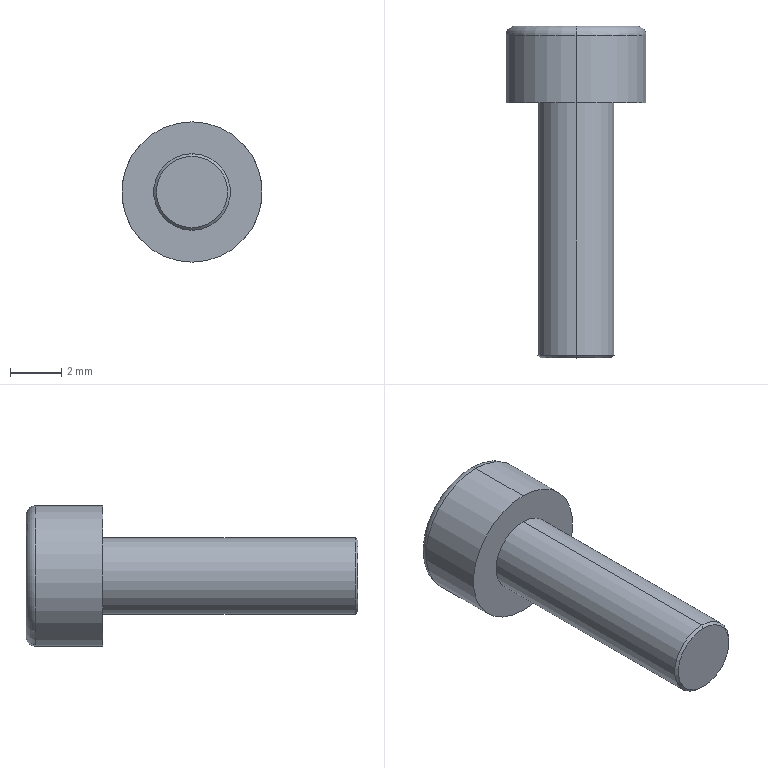Component | SolidWorks | hexagon socket head cap screws gb-1 | 1 solid | 25 faces | box 5.5 x 13 x 5.5 mm | volume 133 mm3 | plane 15 | cone 4 | cylinder 4 | torus 2 | commonest cylinder face diameters 3 x2 5.5 x2
STEP:
#1=CARTESIAN_POINT('',(-3.507,21.249,24.369));
#2=VERTEX_POINT('',#1);
#3=CARTESIAN_POINT('',(-3.507,21.249,24.479));
#4=VERTEX_POINT('',#3);
#5=CARTESIAN_POINT('',(-3.507,21.249,24.424));
#6=DIRECTION('',(0.,-1.,-0.));
#7=DIRECTION('',(0.,0.,-1.));
#8=AXIS2_PLACEMENT_3D('',#5,#6,#7);
#9=CIRCLE('',#8,0.05512);
#10=EDGE_CURVE('',#2,#4,#9,.T.);
#11=ORIENTED_EDGE('',*,*,#10,.F.);
#12=CARTESIAN_POINT('',(-3.507,21.253,24.365));
#13=VERTEX_POINT('',#12);
#14=CARTESIAN_POINT('',(-3.507,21.249,24.369));
#15=DIRECTION('',(-0.,0.7071,-0.7071));
#16=VECTOR('',#15,39.37);
#17=LINE('',#14,#16);
#18=EDGE_CURVE('',#2,#13,#17,.T.);
#19=ORIENTED_EDGE('',*,*,#18,.T.);
#20=CARTESIAN_POINT('',(-3.507,21.253,24.483));
#21=VERTEX_POINT('',#20);
#22=CARTESIAN_POINT('',(-3.507,21.253,24.424));
#23=DIRECTION('',(-0.,1.,0.));
#24=DIRECTION('',(0.,0.,-1.));
#25=AXIS2_PLACEMENT_3D('',#22,#23,#24);
#26=CIRCLE('',#25,0.05906);
#27=EDGE_CURVE('',#21,#13,#26,.T.);
#28=ORIENTED_EDGE('',*,*,#27,.F.);
#29=CARTESIAN_POINT('',(-3.507,21.249,24.479));
#30=DIRECTION('',(0.,0.7071,0.7071));
#31=VECTOR('',#30,39.37);
#32=LINE('',#29,#31);
#33=EDGE_CURVE('',#4,#21,#32,.T.);
#34=ORIENTED_EDGE('',*,*,#33,.F.);
#35=EDGE_LOOP('',(#11,#19,#28,#34));
#36=FACE_OUTER_BOUND('',#35,.T.);
#37=CARTESIAN_POINT('',(-3.507,21.249,24.424));
#38=DIRECTION('',(-0.,1.,0.));
#39=DIRECTION('',(0.,0.,1.));
#40=AXIS2_PLACEMENT_3D('',#37,#38,#39);
#41=CONICAL_SURFACE('',#40,0.05512,0.7854);
#42=ADVANCED_FACE('',(#36),#41,.T.);
#43=CARTESIAN_POINT('',(-3.507,21.761,24.517));
#44=VERTEX_POINT('',#43);
#45=CARTESIAN_POINT('',(-3.507,21.761,24.33));
#46=VERTEX_POINT('',#45);
#47=CARTESIAN_POINT('',(-3.507,21.761,24.424));
#48=DIRECTION('',(-0.,1.,0.));
#49=DIRECTION('',(0.,0.,-1.));
#50=AXIS2_PLACEMENT_3D('',#47,#48,#49);
#51=CIRCLE('',#50,0.0935);
#52=EDGE_CURVE('',#44,#46,#51,.T.);
#53=ORIENTED_EDGE('',*,*,#52,.F.);
#54=CARTESIAN_POINT('',(-3.507,21.746,24.532));
#55=VERTEX_POINT('',#54);
#56=CARTESIAN_POINT('',(-3.507,21.746,24.517));
#57=DIRECTION('',(1.,0.,-0.));
#58=DIRECTION('',(0.,0.,-1.));
#59=AXIS2_PLACEMENT_3D('',#56,#57,#58);
#60=CIRCLE('',#59,0.01476);
#61=EDGE_CURVE('',#44,#55,#60,.T.);
#62=ORIENTED_EDGE('',*,*,#61,.T.);
#63=CARTESIAN_POINT('',(-3.507,21.746,24.315));
#64=VERTEX_POINT('',#63);
#65=CARTESIAN_POINT('',(-3.507,21.746,24.424));
#66=DIRECTION('',(0.,-1.,-0.));
#67=DIRECTION('',(0.,0.,-1.));
#68=AXIS2_PLACEMENT_3D('',#65,#66,#67);
#69=CIRCLE('',#68,0.1083);
#70=EDGE_CURVE('',#64,#55,#69,.T.);
#71=ORIENTED_EDGE('',*,*,#70,.F.);
#72=CARTESIAN_POINT('',(-3.507,21.746,24.33));
#73=DIRECTION('',(-1.,-0.,0.));
#74=DIRECTION('',(0.,0.,1.));
#75=AXIS2_PLACEMENT_3D('',#72,#73,#74);
#76=CIRCLE('',#75,0.01476);
#77=EDGE_CURVE('',#46,#64,#76,.T.);
#78=ORIENTED_EDGE('',*,*,#77,.F.);
#79=EDGE_LOOP('',(#53,#62,#71,#78));
#80=FACE_OUTER_BOUND('',#79,.T.);
#81=CARTESIAN_POINT('',(-3.507,21.746,24.424));
#82=DIRECTION('',(0.,-1.,-0.));
#83=DIRECTION('',(-0.,0.,-1.));
#84=AXIS2_PLACEMENT_3D('',#81,#82,#83);
#85=TOROIDAL_SURFACE('',#84,0.0935,0.01476);
#86=ADVANCED_FACE('',(#80),#85,.T.);
#87=CARTESIAN_POINT('',(-3.507,21.681,24.424));
#88=VERTEX_POINT('',#87);
#89=CARTESIAN_POINT('',(-3.507,21.709,24.473));
#90=VERTEX_POINT('',#89);
#91=CARTESIAN_POINT('',(-3.507,21.709,24.473));
#92=DIRECTION('',(0.,0.5,0.866));
#93=VECTOR('',#92,39.37);
#94=LINE('',#91,#93);
#95=EDGE_CURVE('',#88,#90,#94,.T.);
#96=ORIENTED_EDGE('',*,*,#95,.F.);
#97=CARTESIAN_POINT('',(-3.507,21.709,24.375));
#98=VERTEX_POINT('',#97);
#99=CARTESIAN_POINT('',(-3.507,21.709,24.375));
#100=DIRECTION('',(-0.,0.5,-0.866));
#101=VECTOR('',#100,39.37);
#102=LINE('',#99,#101);
#103=EDGE_CURVE('',#88,#98,#102,.T.);
#104=ORIENTED_EDGE('',*,*,#103,.T.);
#105=CARTESIAN_POINT('',(-3.531,21.709,24.381));
#106=VERTEX_POINT('',#105);
#107=CARTESIAN_POINT('',(-3.507,21.709,24.424));
#108=DIRECTION('',(-0.,1.,0.));
#109=DIRECTION('',(0.,0.,-1.));
#110=AXIS2_PLACEMENT_3D('',#107,#108,#109);
#111=CIRCLE('',#110,0.04921);
#112=EDGE_CURVE('',#98,#106,#111,.T.);
#113=ORIENTED_EDGE('',*,*,#112,.T.);
#114=CARTESIAN_POINT('',(-3.556,21.709,24.424));
#115=VERTEX_POINT('',#114);
#116=CARTESIAN_POINT('',(-3.507,21.709,24.424));
#117=DIRECTION('',(-0.,1.,0.));
#118=DIRECTION('',(0.,0.,-1.));
#119=AXIS2_PLACEMENT_3D('',#116,#117,#118);
#120=CIRCLE('',#119,0.04921);
#121=EDGE_CURVE('',#106,#115,#120,.T.);
#122=ORIENTED_EDGE('',*,*,#121,.T.);
#123=CARTESIAN_POINT('',(-3.531,21.709,24.466));
#124=VERTEX_POINT('',#123);
#125=CARTESIAN_POINT('',(-3.507,21.709,24.424));
#126=DIRECTION('',(-0.,1.,0.));
#127=DIRECTION('',(0.,0.,-1.));
#128=AXIS2_PLACEMENT_3D('',#125,#126,#127);
#129=CIRCLE('',#128,0.04921);
#130=EDGE_CURVE('',#115,#124,#129,.T.);
#131=ORIENTED_EDGE('',*,*,#130,.T.);
#132=CARTESIAN_POINT('',(-3.507,21.709,24.424));
#133=DIRECTION('',(-0.,1.,0.));
#134=DIRECTION('',(-0.,0.,-1.));
#135=AXIS2_PLACEMENT_3D('',#132,#133,#134);
#136=CIRCLE('',#135,0.04921);
#137=EDGE_CURVE('',#124,#90,#136,.T.);
#138=ORIENTED_EDGE('',*,*,#137,.T.);
#139=EDGE_LOOP('',(#96,#104,#113,#122,#131,#138));
#140=FACE_OUTER_BOUND('',#139,.T.);
#141=CARTESIAN_POINT('',(-3.507,21.709,24.424));
#142=DIRECTION('',(-0.,1.,0.));
#143=DIRECTION('',(0.,0.,1.));
#144=AXIS2_PLACEMENT_3D('',#141,#142,#143);
#145=CONICAL_SURFACE('',#144,0.04921,1.047);
#146=ADVANCED_FACE('',(#140),#145,.F.);
#147=ORIENTED_EDGE('',*,*,#27,.T.);
#148=CARTESIAN_POINT('',(-3.507,21.642,24.365));
#149=VERTEX_POINT('',#148);
#150=CARTESIAN_POINT('',(-3.507,21.249,24.365));
#151=DIRECTION('',(-0.,1.,0.));
#152=VECTOR('',#151,39.37);
#153=LINE('',#150,#152);
#154=EDGE_CURVE('',#13,#149,#153,.T.);
#155=ORIENTED_EDGE('',*,*,#154,.T.);
#156=CARTESIAN_POINT('',(-3.507,21.642,24.483));
#157=VERTEX_POINT('',#156);
#158=CARTESIAN_POINT('',(-3.507,21.642,24.424));
#159=DIRECTION('',(0.,-1.,-0.));
#160=DIRECTION('',(0.,0.,-1.));
#161=AXIS2_PLACEMENT_3D('',#158,#159,#160);
#162=CIRCLE('',#161,0.05906);
#163=EDGE_CURVE('',#149,#157,#162,.T.);
#164=ORIENTED_EDGE('',*,*,#163,.T.);
#165=CARTESIAN_POINT('',(-3.507,21.249,24.483));
#166=DIRECTION('',(-0.,1.,0.));
#167=VECTOR('',#166,39.37);
#168=LINE('',#165,#167);
#169=EDGE_CURVE('',#21,#157,#168,.T.);
#170=ORIENTED_EDGE('',*,*,#169,.F.);
#171=EDGE_LOOP('',(#147,#155,#164,#170));
#172=FACE_OUTER_BOUND('',#171,.T.);
#173=CARTESIAN_POINT('',(-3.507,21.249,24.424));
#174=DIRECTION('',(-0.,1.,0.));
#175=DIRECTION('',(0.,0.,1.));
#176=AXIS2_PLACEMENT_3D('',#173,#174,#175);
#177=CYLINDRICAL_SURFACE('',#176,0.05906);
#178=ADVANCED_FACE('',(#172),#177,.T.);
#179=CARTESIAN_POINT('',(-3.507,21.642,24.315));
#180=VERTEX_POINT('',#179);
#181=CARTESIAN_POINT('',(-3.507,21.642,24.532));
#182=VERTEX_POINT('',#181);
#183=CARTESIAN_POINT('',(-3.507,21.642,24.424));
#184=DIRECTION('',(0.,-1.,-0.));
#185=DIRECTION('',(0.,0.,-1.));
#186=AXIS2_PLACEMENT_3D('',#183,#184,#185);
#187=CIRCLE('',#186,0.1083);
#188=EDGE_CURVE('',#180,#182,#187,.T.);
#189=ORIENTED_EDGE('',*,*,#188,.F.);
#190=CARTESIAN_POINT('',(-3.507,21.642,24.315));
#191=DIRECTION('',(-0.,1.,0.));
#192=VECTOR('',#191,39.37);
#193=LINE('',#190,#192);
#194=EDGE_CURVE('',#180,#64,#193,.T.);
#195=ORIENTED_EDGE('',*,*,#194,.T.);
#196=ORIENTED_EDGE('',*,*,#70,.T.);
#197=CARTESIAN_POINT('',(-3.507,21.642,24.532));
#198=DIRECTION('',(-0.,1.,0.));
#199=VECTOR('',#198,39.37);
#200=LINE('',#197,#199);
#201=EDGE_CURVE('',#182,#55,#200,.T.);
#202=ORIENTED_EDGE('',*,*,#201,.F.);
#203=EDGE_LOOP('',(#189,#195,#196,#202));
#204=FACE_OUTER_BOUND('',#203,.T.);
#205=CARTESIAN_POINT('',(-3.507,21.642,24.424));
#206=DIRECTION('',(-0.,1.,0.));
#207=DIRECTION('',(0.,0.,1.));
#208=AXIS2_PLACEMENT_3D('',#205,#206,#207);
#209=CYLINDRICAL_SURFACE('',#208,0.1083);
#210=ADVANCED_FACE('',(#204),#209,.T.);
#211=ORIENTED_EDGE('',*,*,#121,.F.);
#212=CARTESIAN_POINT('',(-3.556,21.709,24.395));
#213=VERTEX_POINT('',#212);
#214=CARTESIAN_POINT('',(-3.556,21.709,24.395));
#215=DIRECTION('',(0.866,0.,-0.5));
#216=VECTOR('',#215,39.37);
#217=LINE('',#214,#216);
#218=EDGE_CURVE('',#213,#106,#217,.T.);
#219=ORIENTED_EDGE('',*,*,#218,.F.);
#220=CARTESIAN_POINT('',(-3.556,21.709,24.452));
#221=DIRECTION('',(0.,0.,-1.));
#222=VECTOR('',#221,39.37);
#223=LINE('',#220,#222);
#224=EDGE_CURVE('',#115,#213,#223,.T.);
#225=ORIENTED_EDGE('',*,*,#224,.F.);
#226=EDGE_LOOP('',(#211,#219,#225));
#227=FACE_OUTER_BOUND('',#226,.T.);
#228=CARTESIAN_POINT('',(-3.507,21.709,24.367));
#229=DIRECTION('',(0.,-1.,-0.));
#230=DIRECTION('',(-0.,0.,-1.));
#231=AXIS2_PLACEMENT_3D('',#228,#229,#230);
#232=PLANE('',#231);
#233=ADVANCED_FACE('',(#227),#232,.F.);
#234=ORIENTED_EDGE('',*,*,#130,.F.);
#235=CARTESIAN_POINT('',(-3.556,21.709,24.452));
#236=VERTEX_POINT('',#235);
#237=CARTESIAN_POINT('',(-3.556,21.709,24.452));
#238=DIRECTION('',(0.,0.,-1.));
#239=VECTOR('',#238,39.37);
#240=LINE('',#237,#239);
#241=EDGE_CURVE('',#236,#115,#240,.T.);
#242=ORIENTED_EDGE('',*,*,#241,.F.);
#243=CARTESIAN_POINT('',(-3.507,21.709,24.481));
#244=DIRECTION('',(-0.866,0.,-0.5));
#245=VECTOR('',#244,39.37);
#246=LINE('',#243,#245);
#247=EDGE_CURVE('',#124,#236,#246,.T.);
#248=ORIENTED_EDGE('',*,*,#247,.F.);
#249=EDGE_LOOP('',(#234,#242,#248));
#250=FACE_OUTER_BOUND('',#249,.T.);
#251=CARTESIAN_POINT('',(-3.507,21.709,24.367));
#252=DIRECTION('',(0.,-1.,-0.));
#253=DIRECTION('',(-0.,0.,-1.));
#254=AXIS2_PLACEMENT_3D('',#251,#252,#253);
#255=PLANE('',#254);
#256=ADVANCED_FACE('',(#250),#255,.F.);
#257=ORIENTED_EDGE('',*,*,#137,.F.);
#258=CARTESIAN_POINT('',(-3.507,21.709,24.481));
#259=VERTEX_POINT('',#258);
#260=CARTESIAN_POINT('',(-3.507,21.709,24.481));
#261=DIRECTION('',(-0.866,0.,-0.5));
#262=VECTOR('',#261,39.37);
#263=LINE('',#260,#262);
#264=EDGE_CURVE('',#259,#124,#263,.T.);
#265=ORIENTED_EDGE('',*,*,#264,.F.);
#266=CARTESIAN_POINT('',(-3.482,21.709,24.466));
#267=VERTEX_POINT('',#266);
#268=CARTESIAN_POINT('',(-3.458,21.709,24.452));
#269=DIRECTION('',(-0.866,-0.,0.5));
#270=VECTOR('',#269,39.37);
#271=LINE('',#268,#270);
#272=EDGE_CURVE('',#267,#259,#271,.T.);
#273=ORIENTED_EDGE('',*,*,#272,.F.);
#274=CARTESIAN_POINT('',(-3.507,21.709,24.424));
#275=DIRECTION('',(-0.,1.,0.));
#276=DIRECTION('',(-0.,0.,-1.));
#277=AXIS2_PLACEMENT_3D('',#274,#275,#276);
#278=CIRCLE('',#277,0.04921);
#279=EDGE_CURVE('',#90,#267,#278,.T.);
#280=ORIENTED_EDGE('',*,*,#279,.F.);
#281=EDGE_LOOP('',(#257,#265,#273,#280));
#282=FACE_OUTER_BOUND('',#281,.T.);
#283=CARTESIAN_POINT('',(-3.507,21.709,24.367));
#284=DIRECTION('',(0.,-1.,-0.));
#285=DIRECTION('',(-0.,0.,-1.));
#286=AXIS2_PLACEMENT_3D('',#283,#284,#285);
#287=PLANE('',#286);
#288=ADVANCED_FACE('',(#282),#287,.F.);
#289=CARTESIAN_POINT('',(-3.458,21.709,24.424));
#290=VERTEX_POINT('',#289);
#291=CARTESIAN_POINT('',(-3.507,21.709,24.424));
#292=DIRECTION('',(-0.,1.,0.));
#293=DIRECTION('',(0.,0.,-1.));
#294=AXIS2_PLACEMENT_3D('',#291,#292,#293);
#295=CIRCLE('',#294,0.04921);
#296=EDGE_CURVE('',#267,#290,#295,.T.);
#297=ORIENTED_EDGE('',*,*,#296,.F.);
#298=CARTESIAN_POINT('',(-3.458,21.709,24.452));
#299=VERTEX_POINT('',#298);
#300=CARTESIAN_POINT('',(-3.458,21.709,24.452));
#301=DIRECTION('',(-0.866,-0.,0.5));
#302=VECTOR('',#301,39.37);
#303=LINE('',#300,#302);
#304=EDGE_CURVE('',#299,#267,#303,.T.);
#305=ORIENTED_EDGE('',*,*,#304,.F.);
#306=CARTESIAN_POINT('',(-3.458,21.709,24.395));
#307=DIRECTION('',(0.,-0.,1.));
#308=VECTOR('',#307,39.37);
#309=LINE('',#306,#308);
#310=EDGE_CURVE('',#290,#299,#309,.T.);
#311=ORIENTED_EDGE('',*,*,#310,.F.);
#312=EDGE_LOOP('',(#297,#305,#311));
#313=FACE_OUTER_BOUND('',#312,.T.);
#314=CARTESIAN_POINT('',(-3.507,21.709,24.367));
#315=DIRECTION('',(0.,-1.,-0.));
#316=DIRECTION('',(-0.,0.,-1.));
#317=AXIS2_PLACEMENT_3D('',#314,#315,#316);
#318=PLANE('',#317);
#319=ADVANCED_FACE('',(#313),#318,.F.);
#320=CARTESIAN_POINT('',(-3.482,21.709,24.381));
#321=VERTEX_POINT('',#320);
#322=CARTESIAN_POINT('',(-3.507,21.709,24.424));
#323=DIRECTION('',(0.,-1.,-0.));
#324=DIRECTION('',(0.,0.,-1.));
#325=AXIS2_PLACEMENT_3D('',#322,#323,#324);
#326=CIRCLE('',#325,0.04921);
#327=EDGE_CURVE('',#321,#290,#326,.T.);
#328=ORIENTED_EDGE('',*,*,#327,.T.);
#329=CARTESIAN_POINT('',(-3.458,21.709,24.395));
#330=VERTEX_POINT('',#329);
#331=CARTESIAN_POINT('',(-3.458,21.709,24.395));
#332=DIRECTION('',(0.,-0.,1.));
#333=VECTOR('',#332,39.37);
#334=LINE('',#331,#333);
#335=EDGE_CURVE('',#330,#290,#334,.T.);
#336=ORIENTED_EDGE('',*,*,#335,.F.);
#337=CARTESIAN_POINT('',(-3.507,21.709,24.367));
#338=DIRECTION('',(0.866,-0.,0.5));
#339=VECTOR('',#338,39.37);
#340=LINE('',#337,#339);
#341=EDGE_CURVE('',#321,#330,#340,.T.);
#342=ORIENTED_EDGE('',*,*,#341,.F.);
#343=EDGE_LOOP('',(#328,#336,#342));
#344=FACE_OUTER_BOUND('',#343,.T.);
#345=CARTESIAN_POINT('',(-3.507,21.709,24.367));
#346=DIRECTION('',(0.,-1.,-0.));
#347=DIRECTION('',(-0.,0.,-1.));
#348=AXIS2_PLACEMENT_3D('',#345,#346,#347);
#349=PLANE('',#348);
#350=ADVANCED_FACE('',(#344),#349,.F.);
#351=CARTESIAN_POINT('',(-3.507,21.709,24.424));
#352=DIRECTION('',(-0.,1.,0.));
#353=DIRECTION('',(-0.,0.,-1.));
#354=AXIS2_PLACEMENT_3D('',#351,#352,#353);
#355=CIRCLE('',#354,0.04921);
#356=EDGE_CURVE('',#321,#98,#355,.T.);
#357=ORIENTED_EDGE('',*,*,#356,.F.);
#358=CARTESIAN_POINT('',(-3.507,21.709,24.367));
#359=VERTEX_POINT('',#358);
#360=CARTESIAN_POINT('',(-3.507,21.709,24.367));
#361=DIRECTION('',(0.866,-0.,0.5));
#362=VECTOR('',#361,39.37);
#363=LINE('',#360,#362);
#364=EDGE_CURVE('',#359,#321,#363,.T.);
#365=ORIENTED_EDGE('',*,*,#364,.F.);
#366=CARTESIAN_POINT('',(-3.556,21.709,24.395));
#367=DIRECTION('',(0.866,0.,-0.5));
#368=VECTOR('',#367,39.37);
#369=LINE('',#366,#368);
#370=EDGE_CURVE('',#106,#359,#369,.T.);
#371=ORIENTED_EDGE('',*,*,#370,.F.);
#372=ORIENTED_EDGE('',*,*,#112,.F.);
#373=EDGE_LOOP('',(#357,#365,#371,#372));
#374=FACE_OUTER_BOUND('',#373,.T.);
#375=CARTESIAN_POINT('',(-3.507,21.709,24.367));
#376=DIRECTION('',(0.,-1.,-0.));
#377=DIRECTION('',(-0.,0.,-1.));
#378=AXIS2_PLACEMENT_3D('',#375,#376,#377);
#379=PLANE('',#378);
#380=ADVANCED_FACE('',(#374),#379,.F.);
#381=CARTESIAN_POINT('',(-3.507,21.761,24.424));
#382=DIRECTION('',(-0.,1.,0.));
#383=DIRECTION('',(0.,0.,-1.));
#384=AXIS2_PLACEMENT_3D('',#381,#382,#383);
#385=CIRCLE('',#384,0.0935);
#386=EDGE_CURVE('',#46,#44,#385,.T.);
#387=ORIENTED_EDGE('',*,*,#386,.T.);
#388=ORIENTED_EDGE('',*,*,#52,.T.);
#389=EDGE_LOOP('',(#387,#388));
#390=FACE_OUTER_BOUND('',#389,.T.);
#391=CARTESIAN_POINT('',(-3.556,21.761,24.395));
#392=VERTEX_POINT('',#391);
#393=CARTESIAN_POINT('',(-3.507,21.761,24.367));
#394=VERTEX_POINT('',#393);
#395=CARTESIAN_POINT('',(-3.556,21.761,24.395));
#396=DIRECTION('',(0.866,0.,-0.5));
#397=VECTOR('',#396,39.37);
#398=LINE('',#395,#397);
#399=EDGE_CURVE('',#392,#394,#398,.T.);
#400=ORIENTED_EDGE('',*,*,#399,.T.);
#401=CARTESIAN_POINT('',(-3.458,21.761,24.395));
#402=VERTEX_POINT('',#401);
#403=CARTESIAN_POINT('',(-3.507,21.761,24.367));
#404=DIRECTION('',(0.866,-0.,0.5));
#405=VECTOR('',#404,39.37);
#406=LINE('',#403,#405);
#407=EDGE_CURVE('',#394,#402,#406,.T.);
#408=ORIENTED_EDGE('',*,*,#407,.T.);
#409=CARTESIAN_POINT('',(-3.458,21.761,24.452));
#410=VERTEX_POINT('',#409);
#411=CARTESIAN_POINT('',(-3.458,21.761,24.395));
#412=DIRECTION('',(0.,-0.,1.));
#413=VECTOR('',#412,39.37);
#414=LINE('',#411,#413);
#415=EDGE_CURVE('',#402,#410,#414,.T.);
#416=ORIENTED_EDGE('',*,*,#415,.T.);
#417=CARTESIAN_POINT('',(-3.507,21.761,24.481));
#418=VERTEX_POINT('',#417);
#419=CARTESIAN_POINT('',(-3.458,21.761,24.452));
#420=DIRECTION('',(-0.866,-0.,0.5));
#421=VECTOR('',#420,39.37);
#422=LINE('',#419,#421);
#423=EDGE_CURVE('',#410,#418,#422,.T.);
#424=ORIENTED_EDGE('',*,*,#423,.T.);
#425=CARTESIAN_POINT('',(-3.556,21.761,24.452));
#426=VERTEX_POINT('',#425);
#427=CARTESIAN_POINT('',(-3.507,21.761,24.481));
#428=DIRECTION('',(-0.866,0.,-0.5));
#429=VECTOR('',#428,39.37);
#430=LINE('',#427,#429);
#431=EDGE_CURVE('',#418,#426,#430,.T.);
#432=ORIENTED_EDGE('',*,*,#431,.T.);
#433=CARTESIAN_POINT('',(-3.556,21.761,24.452));
#434=DIRECTION('',(0.,0.,-1.));
#435=VECTOR('',#434,39.37);
#436=LINE('',#433,#435);
#437=EDGE_CURVE('',#426,#392,#436,.T.);
#438=ORIENTED_EDGE('',*,*,#437,.T.);
#439=EDGE_LOOP('',(#400,#408,#416,#424,#432,#438));
#440=FACE_BOUND('',#439,.T.);
#441=CARTESIAN_POINT('',(-3.507,21.761,24.424));
#442=DIRECTION('',(0.,-1.,-0.));
#443=DIRECTION('',(-0.,0.,-1.));
#444=AXIS2_PLACEMENT_3D('',#441,#442,#443);
#445=PLANE('',#444);
#446=ADVANCED_FACE('',(#390,#440),#445,.F.);
#447=CARTESIAN_POINT('',(-3.507,21.642,24.424));
#448=DIRECTION('',(0.,-1.,-0.));
#449=DIRECTION('',(0.,0.,-1.));
#450=AXIS2_PLACEMENT_3D('',#447,#448,#449);
#451=CIRCLE('',#450,0.1083);
#452=EDGE_CURVE('',#182,#180,#451,.T.);
#453=ORIENTED_EDGE('',*,*,#452,.T.);
#454=ORIENTED_EDGE('',*,*,#188,.T.);
#455=EDGE_LOOP('',(#453,#454));
#456=FACE_OUTER_BOUND('',#455,.T.);
#457=CARTESIAN_POINT('',(-3.507,21.642,24.424));
#458=DIRECTION('',(0.,-1.,-0.));
#459=DIRECTION('',(0.,0.,-1.));
#460=AXIS2_PLACEMENT_3D('',#457,#458,#459);
#461=CIRCLE('',#460,0.05906);
#462=EDGE_CURVE('',#157,#149,#461,.T.);
#463=ORIENTED_EDGE('',*,*,#462,.F.);
#464=ORIENTED_EDGE('',*,*,#163,.F.);
#465=EDGE_LOOP('',(#463,#464));
#466=FACE_BOUND('',#465,.T.);
#467=CARTESIAN_POINT('',(-3.507,21.642,24.424));
#468=DIRECTION('',(0.,-1.,-0.));
#469=DIRECTION('',(-0.,0.,-1.));
#470=AXIS2_PLACEMENT_3D('',#467,#468,#469);
#471=PLANE('',#470);
#472=ADVANCED_FACE('',(#456,#466),#471,.T.);
#473=ORIENTED_EDGE('',*,*,#194,.F.);
#474=ORIENTED_EDGE('',*,*,#452,.F.);
#475=ORIENTED_EDGE('',*,*,#201,.T.);
#476=CARTESIAN_POINT('',(-3.507,21.746,24.424));
#477=DIRECTION('',(0.,-1.,-0.));
#478=DIRECTION('',(0.,0.,-1.));
#479=AXIS2_PLACEMENT_3D('',#476,#477,#478);
#480=CIRCLE('',#479,0.1083);
#481=EDGE_CURVE('',#55,#64,#480,.T.);
#482=ORIENTED_EDGE('',*,*,#481,.T.);
#483=EDGE_LOOP('',(#473,#474,#475,#482));
#484=FACE_OUTER_BOUND('',#483,.T.);
#485=CARTESIAN_POINT('',(-3.507,21.642,24.424));
#486=DIRECTION('',(-0.,1.,0.));
#487=DIRECTION('',(0.,0.,1.));
#488=AXIS2_PLACEMENT_3D('',#485,#486,#487);
#489=CYLINDRICAL_SURFACE('',#488,0.1083);
#490=ADVANCED_FACE('',(#484),#489,.T.);
#491=ORIENTED_EDGE('',*,*,#154,.F.);
#492=CARTESIAN_POINT('',(-3.507,21.253,24.424));
#493=DIRECTION('',(-0.,1.,0.));
#494=DIRECTION('',(0.,0.,-1.));
#495=AXIS2_PLACEMENT_3D('',#492,#493,#494);
#496=CIRCLE('',#495,0.05906);
#497=EDGE_CURVE('',#13,#21,#496,.T.);
#498=ORIENTED_EDGE('',*,*,#497,.T.);
#499=ORIENTED_EDGE('',*,*,#169,.T.);
#500=ORIENTED_EDGE('',*,*,#462,.T.);
#501=EDGE_LOOP('',(#491,#498,#499,#500));
#502=FACE_OUTER_BOUND('',#501,.T.);
#503=CARTESIAN_POINT('',(-3.507,21.249,24.424));
#504=DIRECTION('',(-0.,1.,0.));
#505=DIRECTION('',(0.,0.,1.));
#506=AXIS2_PLACEMENT_3D('',#503,#504,#505);
#507=CYLINDRICAL_SURFACE('',#506,0.05906);
#508=ADVANCED_FACE('',(#502),#507,.T.);
#509=CARTESIAN_POINT('',(-3.507,21.249,24.424));
#510=DIRECTION('',(0.,-1.,-0.));
#511=DIRECTION('',(0.,0.,-1.));
#512=AXIS2_PLACEMENT_3D('',#509,#510,#511);
#513=CIRCLE('',#512,0.05512);
#514=EDGE_CURVE('',#4,#2,#513,.T.);
#515=ORIENTED_EDGE('',*,*,#514,.T.);
#516=ORIENTED_EDGE('',*,*,#10,.T.);
#517=EDGE_LOOP('',(#515,#516));
#518=FACE_OUTER_BOUND('',#517,.T.);
#519=CARTESIAN_POINT('',(-3.507,21.249,24.424));
#520=DIRECTION('',(0.,-1.,-0.));
#521=DIRECTION('',(-0.,0.,-1.));
#522=AXIS2_PLACEMENT_3D('',#519,#520,#521);
#523=PLANE('',#522);
#524=ADVANCED_FACE('',(#518),#523,.T.);
#525=ORIENTED_EDGE('',*,*,#399,.F.);
#526=CARTESIAN_POINT('',(-3.556,21.709,24.395));
#527=DIRECTION('',(-0.,1.,0.));
#528=VECTOR('',#527,39.37);
#529=LINE('',#526,#528);
#530=EDGE_CURVE('',#213,#392,#529,.T.);
#531=ORIENTED_EDGE('',*,*,#530,.F.);
#532=ORIENTED_EDGE('',*,*,#218,.T.);
#533=ORIENTED_EDGE('',*,*,#370,.T.);
#534=CARTESIAN_POINT('',(-3.507,21.709,24.367));
#535=DIRECTION('',(-0.,1.,0.));
#536=VECTOR('',#535,39.37);
#537=LINE('',#534,#536);
#538=EDGE_CURVE('',#359,#394,#537,.T.);
#539=ORIENTED_EDGE('',*,*,#538,.T.);
#540=EDGE_LOOP('',(#525,#531,#532,#533,#539));
#541=FACE_OUTER_BOUND('',#540,.T.);
#542=CARTESIAN_POINT('',(-3.556,21.709,24.395));
#543=DIRECTION('',(0.5,-0.,0.866));
#544=DIRECTION('',(-0.866,-0.,0.5));
#545=AXIS2_PLACEMENT_3D('',#542,#543,#544);
#546=PLANE('',#545);
#547=ADVANCED_FACE('',(#541),#546,.T.);
#548=ORIENTED_EDGE('',*,*,#407,.F.);
#549=ORIENTED_EDGE('',*,*,#538,.F.);
#550=ORIENTED_EDGE('',*,*,#364,.T.);
#551=ORIENTED_EDGE('',*,*,#341,.T.);
#552=CARTESIAN_POINT('',(-3.458,21.709,24.395));
#553=DIRECTION('',(-0.,1.,0.));
#554=VECTOR('',#553,39.37);
#555=LINE('',#552,#554);
#556=EDGE_CURVE('',#330,#402,#555,.T.);
#557=ORIENTED_EDGE('',*,*,#556,.T.);
#558=EDGE_LOOP('',(#548,#549,#550,#551,#557));
#559=FACE_OUTER_BOUND('',#558,.T.);
#560=CARTESIAN_POINT('',(-3.507,21.709,24.367));
#561=DIRECTION('',(-0.5,-0.,0.866));
#562=DIRECTION('',(-0.866,0.,-0.5));
#563=AXIS2_PLACEMENT_3D('',#560,#561,#562);
#564=PLANE('',#563);
#565=ADVANCED_FACE('',(#559),#564,.T.);
#566=ORIENTED_EDGE('',*,*,#415,.F.);
#567=ORIENTED_EDGE('',*,*,#556,.F.);
#568=ORIENTED_EDGE('',*,*,#335,.T.);
#569=ORIENTED_EDGE('',*,*,#310,.T.);
#570=CARTESIAN_POINT('',(-3.458,21.709,24.452));
#571=DIRECTION('',(-0.,1.,0.));
#572=VECTOR('',#571,39.37);
#573=LINE('',#570,#572);
#574=EDGE_CURVE('',#299,#410,#573,.T.);
#575=ORIENTED_EDGE('',*,*,#574,.T.);
#576=EDGE_LOOP('',(#566,#567,#568,#569,#575));
#577=FACE_OUTER_BOUND('',#576,.T.);
#578=CARTESIAN_POINT('',(-3.458,21.709,24.395));
#579=DIRECTION('',(-1.,-0.,0.));
#580=DIRECTION('',(-0.,0.,-1.));
#581=AXIS2_PLACEMENT_3D('',#578,#579,#580);
#582=PLANE('',#581);
#583=ADVANCED_FACE('',(#577),#582,.T.);
#584=ORIENTED_EDGE('',*,*,#423,.F.);
#585=ORIENTED_EDGE('',*,*,#574,.F.);
#586=ORIENTED_EDGE('',*,*,#304,.T.);
#587=ORIENTED_EDGE('',*,*,#272,.T.);
#588=CARTESIAN_POINT('',(-3.507,21.709,24.481));
#589=DIRECTION('',(-0.,1.,0.));
#590=VECTOR('',#589,39.37);
#591=LINE('',#588,#590);
#592=EDGE_CURVE('',#259,#418,#591,.T.);
#593=ORIENTED_EDGE('',*,*,#592,.T.);
#594=EDGE_LOOP('',(#584,#585,#586,#587,#593));
#595=FACE_OUTER_BOUND('',#594,.T.);
#596=CARTESIAN_POINT('',(-3.458,21.709,24.452));
#597=DIRECTION('',(-0.5,0.,-0.866));
#598=DIRECTION('',(0.866,0.,-0.5));
#599=AXIS2_PLACEMENT_3D('',#596,#597,#598);
#600=PLANE('',#599);
#601=ADVANCED_FACE('',(#595),#600,.T.);
#602=ORIENTED_EDGE('',*,*,#431,.F.);
#603=ORIENTED_EDGE('',*,*,#592,.F.);
#604=ORIENTED_EDGE('',*,*,#264,.T.);
#605=ORIENTED_EDGE('',*,*,#247,.T.);
#606=CARTESIAN_POINT('',(-3.556,21.709,24.452));
#607=DIRECTION('',(-0.,1.,0.));
#608=VECTOR('',#607,39.37);
#609=LINE('',#606,#608);
#610=EDGE_CURVE('',#236,#426,#609,.T.);
#611=ORIENTED_EDGE('',*,*,#610,.T.);
#612=EDGE_LOOP('',(#602,#603,#604,#605,#611));
#613=FACE_OUTER_BOUND('',#612,.T.);
#614=CARTESIAN_POINT('',(-3.507,21.709,24.481));
#615=DIRECTION('',(0.5,0.,-0.866));
#616=DIRECTION('',(0.866,-0.,0.5));
#617=AXIS2_PLACEMENT_3D('',#614,#615,#616);
#618=PLANE('',#617);
#619=ADVANCED_FACE('',(#613),#618,.T.);
#620=ORIENTED_EDGE('',*,*,#437,.F.);
#621=ORIENTED_EDGE('',*,*,#610,.F.);
#622=ORIENTED_EDGE('',*,*,#241,.T.);
#623=ORIENTED_EDGE('',*,*,#224,.T.);
#624=ORIENTED_EDGE('',*,*,#530,.T.);
#625=EDGE_LOOP('',(#620,#621,#622,#623,#624));
#626=FACE_OUTER_BOUND('',#625,.T.);
#627=CARTESIAN_POINT('',(-3.556,21.709,24.452));
#628=DIRECTION('',(1.,0.,0.));
#629=DIRECTION('',(-0.,-0.,1.));
#630=AXIS2_PLACEMENT_3D('',#627,#628,#629);
#631=PLANE('',#630);
#632=ADVANCED_FACE('',(#626),#631,.T.);
#633=ORIENTED_EDGE('',*,*,#103,.F.);
#634=ORIENTED_EDGE('',*,*,#95,.T.);
#635=ORIENTED_EDGE('',*,*,#279,.T.);
#636=ORIENTED_EDGE('',*,*,#296,.T.);
#637=ORIENTED_EDGE('',*,*,#327,.F.);
#638=ORIENTED_EDGE('',*,*,#356,.T.);
#639=EDGE_LOOP('',(#633,#634,#635,#636,#637,#638));
#640=FACE_OUTER_BOUND('',#639,.T.);
#641=CARTESIAN_POINT('',(-3.507,21.709,24.424));
#642=DIRECTION('',(-0.,1.,0.));
#643=DIRECTION('',(0.,0.,1.));
#644=AXIS2_PLACEMENT_3D('',#641,#642,#643);
#645=CONICAL_SURFACE('',#644,0.04921,1.047);
#646=ADVANCED_FACE('',(#640),#645,.F.);
#647=ORIENTED_EDGE('',*,*,#61,.F.);
#648=ORIENTED_EDGE('',*,*,#386,.F.);
#649=ORIENTED_EDGE('',*,*,#77,.T.);
#650=ORIENTED_EDGE('',*,*,#481,.F.);
#651=EDGE_LOOP('',(#647,#648,#649,#650));
#652=FACE_OUTER_BOUND('',#651,.T.);
#653=CARTESIAN_POINT('',(-3.507,21.746,24.424));
#654=DIRECTION('',(0.,-1.,-0.));
#655=DIRECTION('',(-0.,0.,-1.));
#656=AXIS2_PLACEMENT_3D('',#653,#654,#655);
#657=TOROIDAL_SURFACE('',#656,0.0935,0.01476);
#658=ADVANCED_FACE('',(#652),#657,.T.);
#659=ORIENTED_EDGE('',*,*,#18,.F.);
#660=ORIENTED_EDGE('',*,*,#514,.F.);
#661=ORIENTED_EDGE('',*,*,#33,.T.);
#662=ORIENTED_EDGE('',*,*,#497,.F.);
#663=EDGE_LOOP('',(#659,#660,#661,#662));
#664=FACE_OUTER_BOUND('',#663,.T.);
#665=CARTESIAN_POINT('',(-3.507,21.249,24.424));
#666=DIRECTION('',(-0.,1.,0.));
#667=DIRECTION('',(0.,0.,1.));
#668=AXIS2_PLACEMENT_3D('',#665,#666,#667);
#669=CONICAL_SURFACE('',#668,0.05512,0.7854);
#670=ADVANCED_FACE('',(#664),#669,.T.);
#671=CLOSED_SHELL('',(#42,#86,#146,#178,#210,#233,#256,#288,#319,#350,#380,#446,#472,#490,#508,#524,#547,#565,#583,#601,#619,#632,#646,#658,#670));
#672=MANIFOLD_SOLID_BREP('',#671);
#673=CARTESIAN_POINT('',(0.,0.,0.));
#674=DIRECTION('',(0.,0.,1.));
#675=DIRECTION('',(1.,0.,0.));
#676=AXIS2_PLACEMENT_3D('',#673,#674,#675);
#677=(LENGTH_UNIT()NAMED_UNIT(*)SI_UNIT($,.METRE.));
#678=LENGTH_MEASURE_WITH_UNIT(LENGTH_MEASURE(0.0254),#677);
#679=DIMENSIONAL_EXPONENTS(1.,0.,0.,0.,0.,0.,0.);
#680=(CONVERSION_BASED_UNIT('',#678)LENGTH_UNIT()NAMED_UNIT(#679));
#681=UNCERTAINTY_MEASURE_WITH_UNIT(LENGTH_MEASURE(0.00001),#680,'','');
#682=(NAMED_UNIT(*)PLANE_ANGLE_UNIT()SI_UNIT($,.RADIAN.));
#683=(NAMED_UNIT(*)SI_UNIT($,.STERADIAN.)SOLID_ANGLE_UNIT());
#684=(GEOMETRIC_REPRESENTATION_CONTEXT(3)GLOBAL_UNCERTAINTY_ASSIGNED_CONTEXT((#681))GLOBAL_UNIT_ASSIGNED_CONTEXT((#680,#682,#683))REPRESENTATION_CONTEXT('',''));
#685=ADVANCED_BREP_SHAPE_REPRESENTATION('',(#672,#676),#684);
#686=COLOUR_RGB('',0.7922,0.8196,0.9333);
#687=FILL_AREA_STYLE_COLOUR('',#686);
#688=FILL_AREA_STYLE('',(#687));
#689=SURFACE_STYLE_FILL_AREA(#688);
#690=SURFACE_SIDE_STYLE('',(#689));
#691=SURFACE_STYLE_USAGE(.BOTH.,#690);
#692=PRESENTATION_STYLE_ASSIGNMENT((#691));
#693=STYLED_ITEM('',(#692),#672);
#694=PRESENTATION_LAYER_ASSIGNMENT('','',(#693));
#695=(LENGTH_UNIT()NAMED_UNIT(*)SI_UNIT($,.METRE.));
#696=LENGTH_MEASURE_WITH_UNIT(LENGTH_MEASURE(0.0254),#695);
#697=DIMENSIONAL_EXPONENTS(1.,0.,0.,0.,0.,0.,0.);
#698=(CONVERSION_BASED_UNIT('',#696)LENGTH_UNIT()NAMED_UNIT(#697));
#699=UNCERTAINTY_MEASURE_WITH_UNIT(LENGTH_MEASURE(0.00001),#698,'','');
#700=(NAMED_UNIT(*)PLANE_ANGLE_UNIT()SI_UNIT($,.RADIAN.));
#701=(NAMED_UNIT(*)SI_UNIT($,.STERADIAN.)SOLID_ANGLE_UNIT());
#702=(GEOMETRIC_REPRESENTATION_CONTEXT(3)GLOBAL_UNCERTAINTY_ASSIGNED_CONTEXT((#699))GLOBAL_UNIT_ASSIGNED_CONTEXT((#698,#700,#701))REPRESENTATION_CONTEXT('',''));
#703=MECHANICAL_DESIGN_GEOMETRIC_PRESENTATION_REPRESENTATION('',(#693),#702);